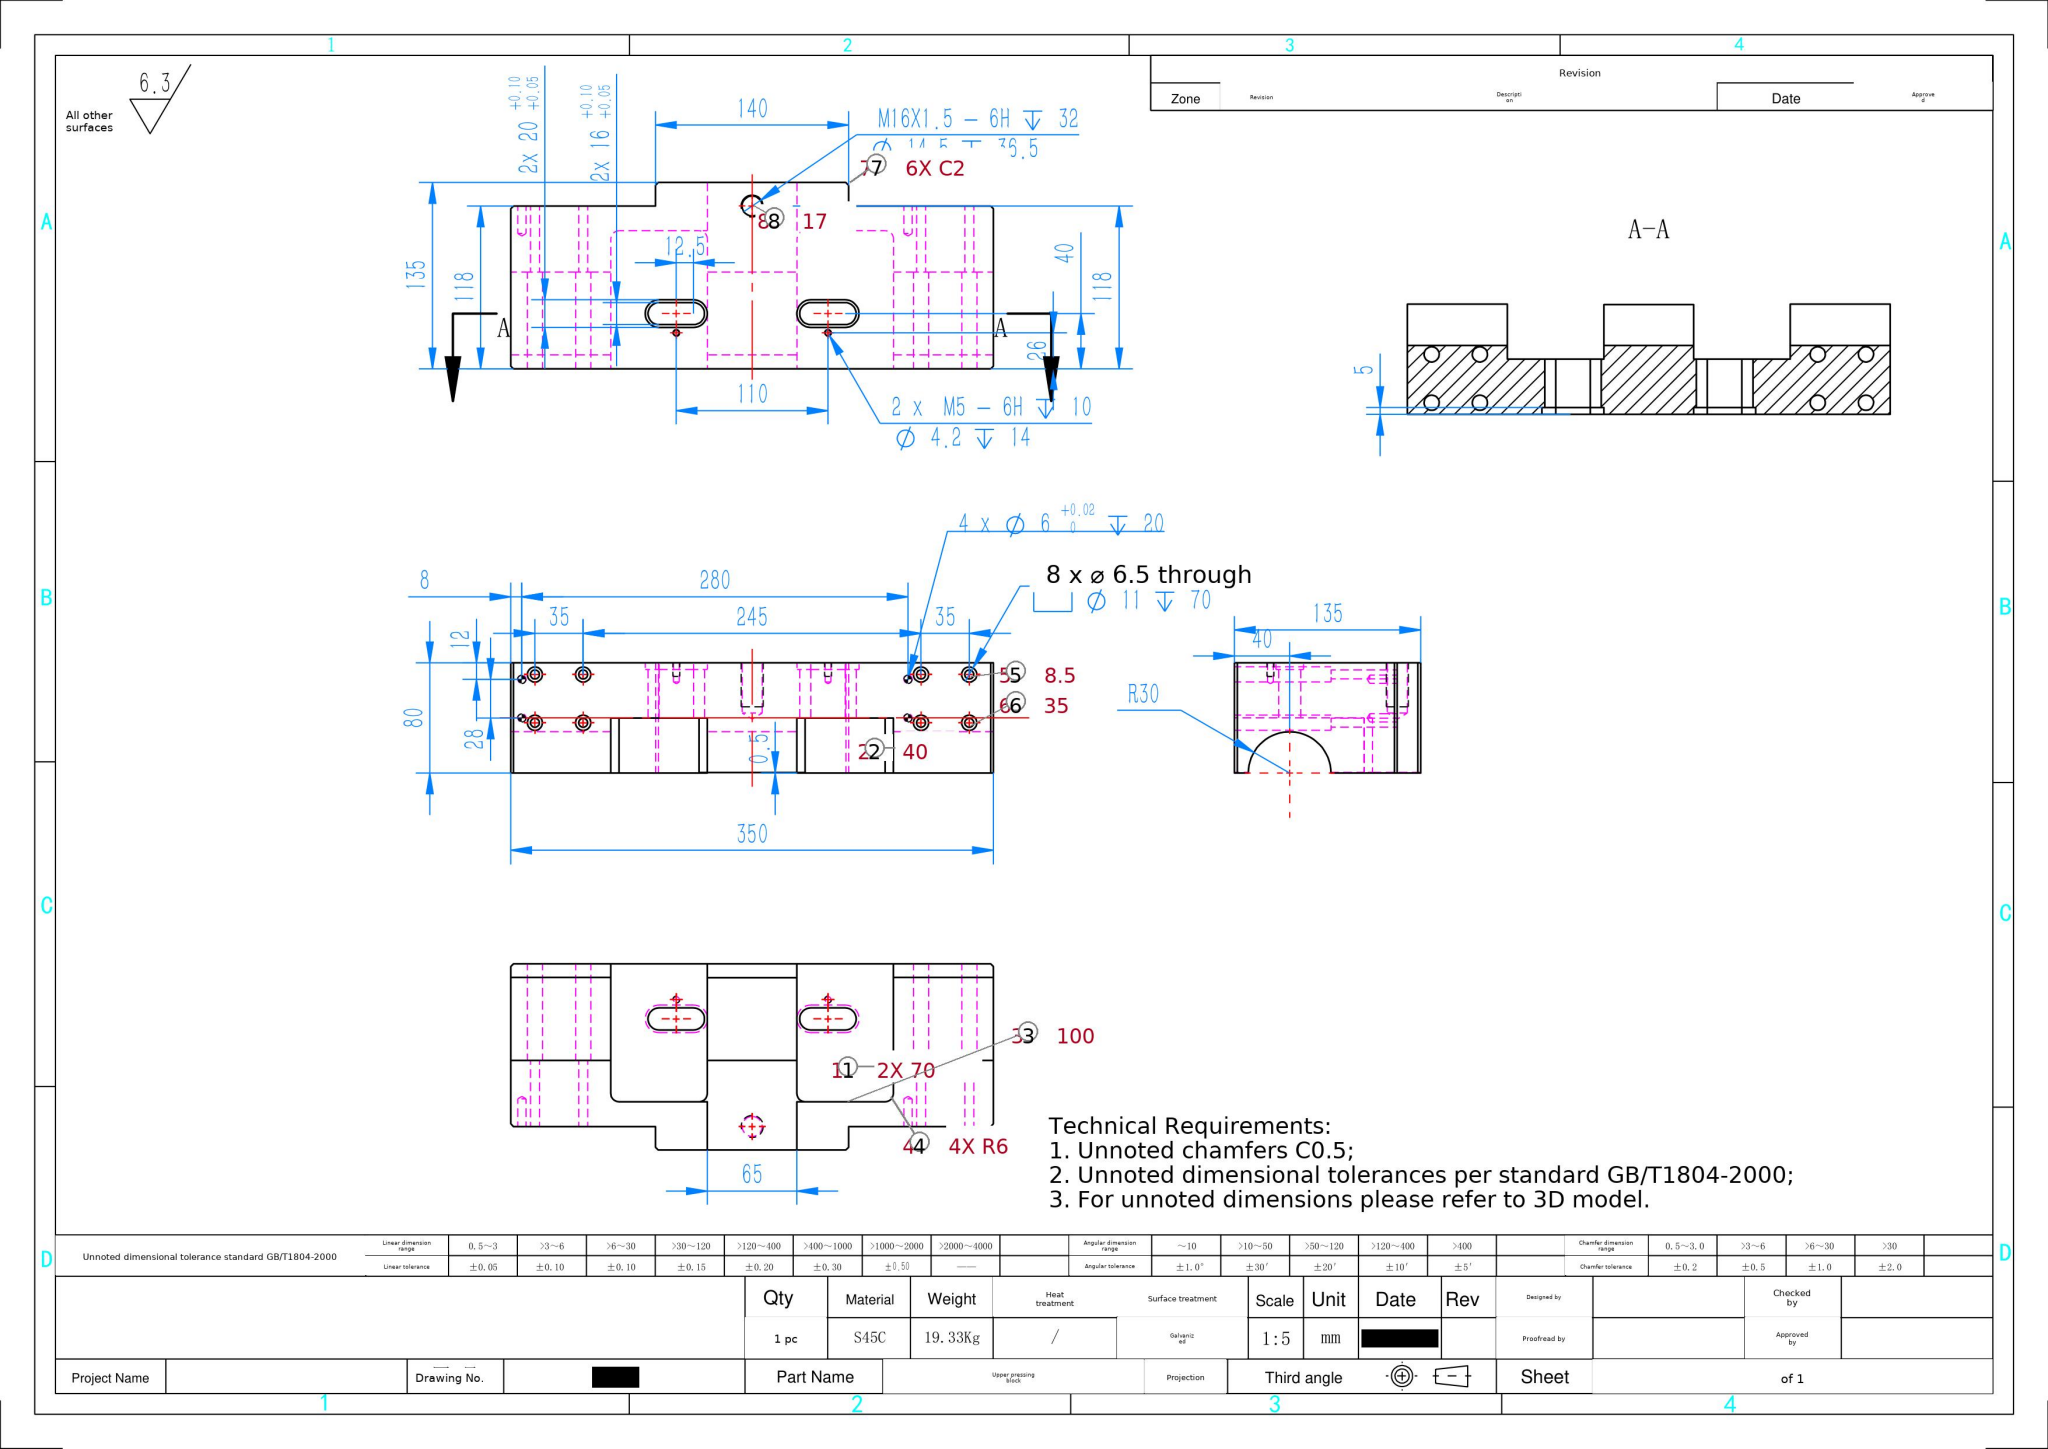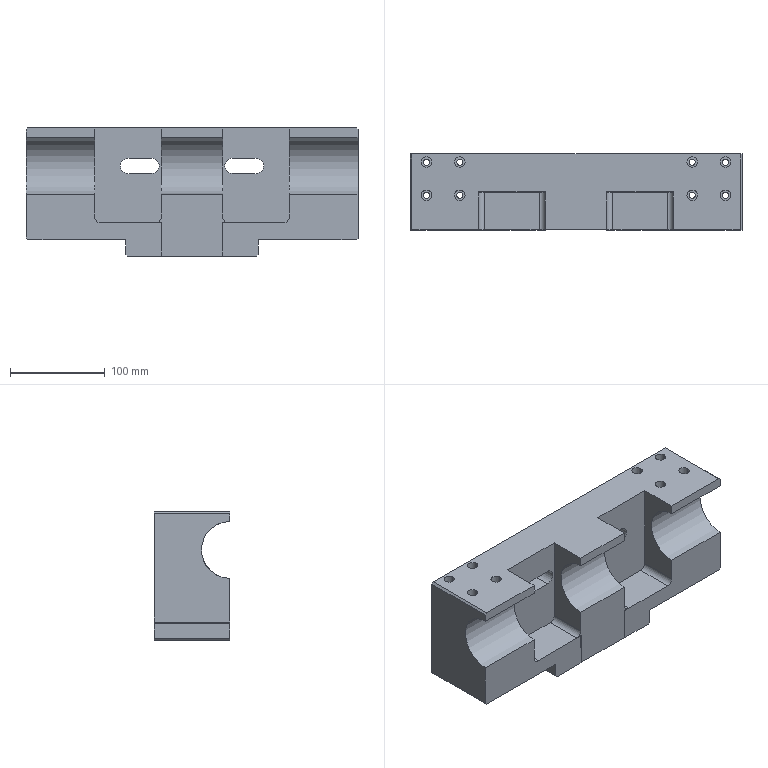Part | SolidWorks | mm | material S45C | 1 solid | 124 faces | box 350 x 80 x 135 mm | volume 2510177 mm3 | cylinder 61 | plane 49 | cone 14 | commonest cylinder face diameters 11 x16 6.5 x16 6 x8 4.2 x4 16 x4 12 x4 20 x4 60 x3
build123d program:
from build123d import *

# Parameters (mm, degrees)
SKETCH1_W                                       = 350
SKETCH1_H                                       = 80
BOSS_EXTRUDE1_DEPTH                             = 100
SKETCH2_R                                       = 30
CUT_EXTRUDE1_DEPTH                              = 367.197
SKETCH3_W                                       = 70
SKETCH3_H                                       = 40
CUT_EXTRUDE2_DEPTH                              = 206.487
CUT_EXTRUDE3_DEPTH                              = 217.852
SKETCH5_W                                       = 140
SKETCH5_H                                       = 80
BOSS_EXTRUDE2_DEPTH                             = 35
SKETCH6_W                                       = 105
SKETCH6_H                                       = 80
SKETCH6_W_2                                     = 32.5
SKETCH6_H_2                                     = 40
BOSS_EXTRUDE3_DEPTH                             = 18
SKETCH7_W                                       = 65
SKETCH7_H                                       = 135
CUT_EXTRUDE4_DEPTH                              = 0.5
FILLET1_R                                       = 6
M5_TAPPED_HOLE7_D                               = 4.2
M5_TAPPED_HOLE7_DEPTH                           = 14
M5_TAPPED_HOLE7_TIP                             = 1.262
M6_HEX_SOCKET_HEAD_CAP_SCREW_CBORE1_D           = 6.5
M6_HEX_SOCKET_HEAD_CAP_SCREW_CBORE1_CBORE_D     = 11
M6_HEX_SOCKET_HEAD_CAP_SCREW_CBORE1_CBORE_DEPTH = 70
F_6_0MM_DOWEL_PIN_HOLE1_D                       = 6
F_6_0MM_DOWEL_PIN_HOLE1_DEPTH                   = 20
F_6_0MM_DOWEL_PIN_HOLE1_TIP                     = 1.803
CUT_EXTRUDE5_DEPTH                              = 5
M16X1_5_TAPPED_HOLE1_D                          = 14.5
M16X1_5_TAPPED_HOLE1_DEPTH                      = 36.5
M16X1_5_TAPPED_HOLE1_TIP                        = 4.356
CHAMFER1_SIZE                                   = 2


with BuildPart() as part:
    # Sketch1 → Boss-Extrude1 (new body)
    with BuildSketch(Plane.XY):
        Rectangle(SKETCH1_W, SKETCH1_H)
    extrude(amount=BOSS_EXTRUDE1_DEPTH)

    # Sketch2 → Cut-Extrude1 (cut, through all)
    with BuildSketch(Plane(origin=(175, 0, 0), x_dir=(0, 0, -1), z_dir=(1, 0, 0))):
        with Locations((-60, -40)):
            Circle(SKETCH2_R)
    extrude(amount=-CUT_EXTRUDE1_DEPTH, mode=Mode.SUBTRACT)

    # Sketch3 → Cut-Extrude2 (cut, through all)
    with BuildSketch(Plane.XY.offset(100)):
        with Locations((-67.5, -20)):
            Rectangle(SKETCH3_W, SKETCH3_H)
        with Locations((67.5, -20)):
            Rectangle(SKETCH3_W, SKETCH3_H)
    extrude(amount=-CUT_EXTRUDE2_DEPTH, mode=Mode.SUBTRACT)

    # Sketch4 → Cut-Extrude3 (cut, through all)
    with BuildSketch(Plane(origin=(0, 40, 0), x_dir=(1, 0, 0), z_dir=(0, 1, 0))):
        with BuildLine():
            Line((-67.5, -52), (-42.5, -52))
            ThreePointArc((-42.5, -52), (-34.5, -60), (-42.5, -68))
            Line((-42.5, -68), (-67.5, -68))
            ThreePointArc((-67.5, -68), (-75.5, -60), (-67.5, -52))
        make_face()
        with BuildLine():
            Line((42.5, -52), (67.5, -52))
            ThreePointArc((67.5, -52), (75.5, -60), (67.5, -68))
            Line((67.5, -68), (42.5, -68))
            ThreePointArc((42.5, -68), (34.5, -60), (42.5, -52))
        make_face()
    extrude(amount=-CUT_EXTRUDE3_DEPTH, mode=Mode.SUBTRACT)

    # Sketch5 → Boss-Extrude2 (add)
    with BuildSketch(Plane(origin=(0, 0, 0), x_dir=(-1, 0, 0), z_dir=(0, 0, -1))):
        Rectangle(SKETCH5_W, SKETCH5_H)
    extrude(amount=BOSS_EXTRUDE2_DEPTH)

    # Sketch6 → Boss-Extrude3 (add)
    with BuildSketch(Plane(origin=(0, 0, 0), x_dir=(-1, 0, 0), z_dir=(0, 0, -1))):
        Polygon((-102.5, 0), (-70, 0), (-70, 40), (-175, 40), (-175, -40), (-102.5, -40), align=None)
        with Locations((122.5, 0)):
            Rectangle(SKETCH6_W, SKETCH6_H)
        with Locations((-86.25, -20)):
            Rectangle(SKETCH6_W_2, SKETCH6_H_2)
    extrude(amount=BOSS_EXTRUDE3_DEPTH)

    # Sketch7 → Cut-Extrude4 (cut)
    with BuildSketch(Plane.XZ.offset(40)):
        with Locations((0, 32.5)):
            Rectangle(SKETCH7_W, SKETCH7_H)
    extrude(amount=-CUT_EXTRUDE4_DEPTH, mode=Mode.SUBTRACT)

    # Fillet1
    fillet1_edges = [part.edges().sort_by_distance(p)[0] for p in [
        (-32.5, -19.75, 0),
        (-102.5, -20, 0),
        (32.5, -19.75, 0),
        (102.5, -20, 0),
    ]]
    fillet(fillet1_edges, radius=FILLET1_R)

    # M5 Tapped Hole7
    with Locations(Plane(origin=(0, 40, 0), x_dir=(1, 0, 0), z_dir=(0, 1, 0))):
        with Locations((-55, -74), (55, -74)):
            Hole(M5_TAPPED_HOLE7_D / 2, depth=M5_TAPPED_HOLE7_DEPTH)
            with Locations((0, 0, -(M5_TAPPED_HOLE7_DEPTH + M5_TAPPED_HOLE7_TIP / 2))):  # 118° drill point
                Cone(0, M5_TAPPED_HOLE7_D / 2, M5_TAPPED_HOLE7_TIP, mode=Mode.SUBTRACT)

    # M6 Hex Socket Head Cap Screw CBORE1 (through all)
    with Locations(Plane.XY.offset(100)):
        with Locations((-122.5, -3.5), (-122.5, 31.5), (-157.5, -3.5), (-157.5, 31.5), (157.5, -3.5), (157.5, 31.5), (122.5, -3.5), (122.5, 31.5)):
            CounterBoreHole(M6_HEX_SOCKET_HEAD_CAP_SCREW_CBORE1_D / 2, M6_HEX_SOCKET_HEAD_CAP_SCREW_CBORE1_CBORE_D / 2, M6_HEX_SOCKET_HEAD_CAP_SCREW_CBORE1_CBORE_DEPTH)

    # 6.0mm Dowel Pin Hole1
    with Locations(Plane(origin=(0, 0, -18), x_dir=(-1, 0, 0), z_dir=(0, 0, -1))):
        with Locations((167, 28), (167, 0), (-113, 28), (-113, 0)):
            Hole(F_6_0MM_DOWEL_PIN_HOLE1_D / 2, depth=F_6_0MM_DOWEL_PIN_HOLE1_DEPTH)
            with Locations((0, 0, -(F_6_0MM_DOWEL_PIN_HOLE1_DEPTH + F_6_0MM_DOWEL_PIN_HOLE1_TIP / 2))):  # 118° drill point
                Cone(0, F_6_0MM_DOWEL_PIN_HOLE1_D / 2, F_6_0MM_DOWEL_PIN_HOLE1_TIP, mode=Mode.SUBTRACT)

    # Sketch23 → Cut-Extrude5 (cut)
    with BuildSketch(Plane(origin=(0, 40, 0), x_dir=(1, 0, 0), z_dir=(0, 1, 0))):
        with BuildLine():
            Line((-67.5, -70), (-42.5, -70))
            ThreePointArc((-42.5, -70), (-32.5, -60), (-42.5, -50))
            Line((-42.5, -50), (-67.5, -50))
            ThreePointArc((-67.5, -50), (-77.5, -60), (-67.5, -70))
        make_face()
        with BuildLine():
            Line((42.5, -70), (67.5, -70))
            ThreePointArc((67.5, -70), (77.5, -60), (67.5, -50))
            Line((67.5, -50), (42.5, -50))
            ThreePointArc((42.5, -50), (32.5, -60), (42.5, -70))
        make_face()
    extrude(amount=-CUT_EXTRUDE5_DEPTH, mode=Mode.SUBTRACT)

    # M16x1.5 Tapped Hole1
    with Locations(Plane(origin=(0, 40, 0), x_dir=(1, 0, 0), z_dir=(0, 1, 0))):
        with Locations((0, 18)):
            Hole(M16X1_5_TAPPED_HOLE1_D / 2, depth=M16X1_5_TAPPED_HOLE1_DEPTH)
            with Locations((0, 0, -(M16X1_5_TAPPED_HOLE1_DEPTH + M16X1_5_TAPPED_HOLE1_TIP / 2))):  # 118° drill point
                Cone(0, M16X1_5_TAPPED_HOLE1_D / 2, M16X1_5_TAPPED_HOLE1_TIP, mode=Mode.SUBTRACT)

    # Chamfer1
    chamfer1_edges = [part.edges().sort_by_distance(p)[0] for p in [
        (70, 0, -35),
        (-70, 0, -35),
        (-175, 0, 100),
        (-175, 0, -18),
        (175, 0, -18),
        (175, 0, 100),
    ]]
    chamfer(chamfer1_edges, length=CHAMFER1_SIZE)


solid = part.part